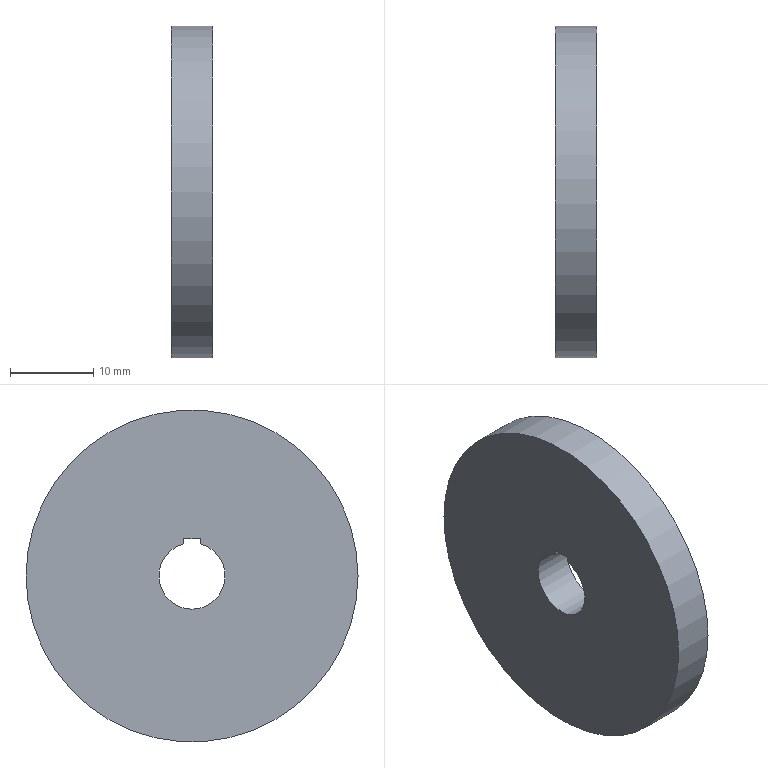Component | NX | SHE_JI-6 | 1 solid | 7 faces | box 5 x 40 x 40 mm | volume 6026 mm3 | plane 5 | cylinder 2 | commonest cylinder face diameters 40 x1 8 x1
STEP:
#1=CARTESIAN_POINT('',(0.,0.,0.));
#2=DIRECTION('',(0.,0.,1.));
#3=DIRECTION('',(1.,0.,0.));
#4=AXIS2_PLACEMENT_3D('',#1,#2,#3);
#5=CARTESIAN_POINT('',(-21.06,-1.,40.5));
#6=VERTEX_POINT('',#5);
#7=CARTESIAN_POINT('',(-21.06,-1.,39.873));
#8=VERTEX_POINT('',#7);
#9=CARTESIAN_POINT('',(-21.06,-1.,36.));
#10=DIRECTION('',(0.,-0.,-1.));
#11=VECTOR('',#10,1.);
#12=LINE('',#9,#11);
#13=CARTESIAN_POINT('',(-21.06,-0.,36.));
#14=DIRECTION('',(1.,0.,0.));
#15=DIRECTION('',(0.,1.,0.));
#16=AXIS2_PLACEMENT_3D('',#13,#14,#15);
#17=PLANE('',#16);
#18=CARTESIAN_POINT('',(-1.,0.));
#19=DIRECTION('',(-0.,-1.));
#20=VECTOR('',#19,1.);
#21=LINE('',#18,#20);
#22=(GEOMETRIC_REPRESENTATION_CONTEXT(2)PARAMETRIC_REPRESENTATION_CONTEXT()REPRESENTATION_CONTEXT('',''));
#23=DEFINITIONAL_REPRESENTATION('',(#21),#22);
#24=PCURVE('',#17,#23);
#25=CARTESIAN_POINT('',(-31.06,-1.,40.5));
#26=DIRECTION('',(0.,-1.,0.));
#27=DIRECTION('',(0.,-0.,-1.));
#28=AXIS2_PLACEMENT_3D('',#25,#26,#27);
#29=PLANE('',#28);
#30=CARTESIAN_POINT('',(4.5,10.));
#31=DIRECTION('',(1.,0.));
#32=VECTOR('',#31,1.);
#33=LINE('',#30,#32);
#34=(GEOMETRIC_REPRESENTATION_CONTEXT(2)PARAMETRIC_REPRESENTATION_CONTEXT()REPRESENTATION_CONTEXT('',''));
#35=DEFINITIONAL_REPRESENTATION('',(#33),#34);
#36=PCURVE('',#29,#35);
#37=SURFACE_CURVE('',#12,(#24,#36),.PCURVE_S1.);
#38=EDGE_CURVE('',#6,#8,#37,.T.);
#39=ORIENTED_EDGE('',*,*,#38,.F.);
#40=CARTESIAN_POINT('',(-21.06,1.,40.5));
#41=VERTEX_POINT('',#40);
#42=CARTESIAN_POINT('',(-21.06,-0.,40.5));
#43=DIRECTION('',(0.,-1.,-0.));
#44=VECTOR('',#43,1.);
#45=LINE('',#42,#44);
#46=CARTESIAN_POINT('',(-0.,4.5));
#47=DIRECTION('',(-1.,-0.));
#48=VECTOR('',#47,1.);
#49=LINE('',#46,#48);
#50=(GEOMETRIC_REPRESENTATION_CONTEXT(2)PARAMETRIC_REPRESENTATION_CONTEXT()REPRESENTATION_CONTEXT('',''));
#51=DEFINITIONAL_REPRESENTATION('',(#49),#50);
#52=PCURVE('',#17,#51);
#53=CARTESIAN_POINT('',(-31.06,1.,40.5));
#54=DIRECTION('',(0.,-0.,1.));
#55=DIRECTION('',(0.,-1.,-0.));
#56=AXIS2_PLACEMENT_3D('',#53,#54,#55);
#57=PLANE('',#56);
#58=CARTESIAN_POINT('',(1.,10.));
#59=DIRECTION('',(1.,0.));
#60=VECTOR('',#59,1.);
#61=LINE('',#58,#60);
#62=(GEOMETRIC_REPRESENTATION_CONTEXT(2)PARAMETRIC_REPRESENTATION_CONTEXT()REPRESENTATION_CONTEXT('',''));
#63=DEFINITIONAL_REPRESENTATION('',(#61),#62);
#64=PCURVE('',#57,#63);
#65=SURFACE_CURVE('',#45,(#52,#64),.PCURVE_S1.);
#66=EDGE_CURVE('',#41,#6,#65,.T.);
#67=ORIENTED_EDGE('',*,*,#66,.F.);
#68=CARTESIAN_POINT('',(-21.06,1.,39.873));
#69=VERTEX_POINT('',#68);
#70=CARTESIAN_POINT('',(-21.06,1.,36.));
#71=DIRECTION('',(0.,0.,1.));
#72=VECTOR('',#71,1.);
#73=LINE('',#70,#72);
#74=CARTESIAN_POINT('',(1.,0.));
#75=DIRECTION('',(0.,1.));
#76=VECTOR('',#75,1.);
#77=LINE('',#74,#76);
#78=(GEOMETRIC_REPRESENTATION_CONTEXT(2)PARAMETRIC_REPRESENTATION_CONTEXT()REPRESENTATION_CONTEXT('',''));
#79=DEFINITIONAL_REPRESENTATION('',(#77),#78);
#80=PCURVE('',#17,#79);
#81=CARTESIAN_POINT('',(-31.06,1.,36.7));
#82=DIRECTION('',(0.,1.,0.));
#83=DIRECTION('',(-1.,0.,0.));
#84=AXIS2_PLACEMENT_3D('',#81,#82,#83);
#85=PLANE('',#84);
#86=CARTESIAN_POINT('',(-10.,-0.7));
#87=DIRECTION('',(0.,1.));
#88=VECTOR('',#87,1.);
#89=LINE('',#86,#88);
#90=(GEOMETRIC_REPRESENTATION_CONTEXT(2)PARAMETRIC_REPRESENTATION_CONTEXT()REPRESENTATION_CONTEXT('',''));
#91=DEFINITIONAL_REPRESENTATION('',(#89),#90);
#92=PCURVE('',#85,#91);
#93=SURFACE_CURVE('',#73,(#80,#92),.PCURVE_S1.);
#94=EDGE_CURVE('',#69,#41,#93,.T.);
#95=ORIENTED_EDGE('',*,*,#94,.F.);
#96=CARTESIAN_POINT('',(-21.06,-0.,36.));
#97=DIRECTION('',(-1.,0.,0.));
#98=DIRECTION('',(0.,1.,-0.));
#99=AXIS2_PLACEMENT_3D('',#96,#97,#98);
#100=CIRCLE('',#99,4.);
#101=CARTESIAN_POINT('',(4.,-0.));
#102=CARTESIAN_POINT('',(4.,-6.928));
#103=CARTESIAN_POINT('',(-2.,-3.464));
#104=CARTESIAN_POINT('',(-8.,-0.));
#105=CARTESIAN_POINT('',(-2.,3.464));
#106=CARTESIAN_POINT('',(4.,6.928));
#107=CARTESIAN_POINT('',(4.,-0.));
#108=(BOUNDED_CURVE()B_SPLINE_CURVE(2,(#101,#102,#103,#104,#105,#106,#107),.UNSPECIFIED.,.T.,.F.)B_SPLINE_CURVE_WITH_KNOTS((1,2,2,2,2,1),(-2.094,0.,2.094,4.189,6.283,8.378),.UNSPECIFIED.)CURVE()GEOMETRIC_REPRESENTATION_ITEM()RATIONAL_B_SPLINE_CURVE((1.,0.5,1.,0.5,1.,0.5,1.))REPRESENTATION_ITEM(''));
#109=(GEOMETRIC_REPRESENTATION_CONTEXT(2)PARAMETRIC_REPRESENTATION_CONTEXT()REPRESENTATION_CONTEXT('',''));
#110=DEFINITIONAL_REPRESENTATION('',(#108),#109);
#111=PCURVE('',#17,#110);
#112=CARTESIAN_POINT('',(-21.06,-0.,36.));
#113=DIRECTION('',(-1.,0.,0.));
#114=DIRECTION('',(0.,1.,-0.));
#115=AXIS2_PLACEMENT_3D('',#112,#113,#114);
#116=CYLINDRICAL_SURFACE('',#115,4.);
#117=CARTESIAN_POINT('',(-6.283,0.));
#118=DIRECTION('',(1.,0.));
#119=VECTOR('',#118,1.);
#120=LINE('',#117,#119);
#121=(GEOMETRIC_REPRESENTATION_CONTEXT(2)PARAMETRIC_REPRESENTATION_CONTEXT()REPRESENTATION_CONTEXT('',''));
#122=DEFINITIONAL_REPRESENTATION('',(#120),#121);
#123=PCURVE('',#116,#122);
#124=SURFACE_CURVE('',#100,(#111,#123),.PCURVE_S1.);
#125=EDGE_CURVE('',#69,#8,#124,.T.);
#126=ORIENTED_EDGE('',*,*,#125,.T.);
#127=EDGE_LOOP('',(#39,#67,#95,#126));
#128=FACE_BOUND('',#127,.T.);
#129=CARTESIAN_POINT('',(-21.06,20.,36.));
#130=VERTEX_POINT('',#129);
#131=CARTESIAN_POINT('',(-21.06,-0.,36.));
#132=DIRECTION('',(-1.,0.,0.));
#133=DIRECTION('',(0.,1.,0.));
#134=AXIS2_PLACEMENT_3D('',#131,#132,#133);
#135=CIRCLE('',#134,20.);
#136=CARTESIAN_POINT('',(20.,0.));
#137=CARTESIAN_POINT('',(20.,-34.641));
#138=CARTESIAN_POINT('',(-10.,-17.321));
#139=CARTESIAN_POINT('',(-40.,-0.));
#140=CARTESIAN_POINT('',(-10.,17.321));
#141=CARTESIAN_POINT('',(20.,34.641));
#142=CARTESIAN_POINT('',(20.,0.));
#143=(BOUNDED_CURVE()B_SPLINE_CURVE(2,(#136,#137,#138,#139,#140,#141,#142),.UNSPECIFIED.,.T.,.F.)B_SPLINE_CURVE_WITH_KNOTS((1,2,2,2,2,1),(-2.094,0.,2.094,4.189,6.283,8.378),.UNSPECIFIED.)CURVE()GEOMETRIC_REPRESENTATION_ITEM()RATIONAL_B_SPLINE_CURVE((1.,0.5,1.,0.5,1.,0.5,1.))REPRESENTATION_ITEM(''));
#144=(GEOMETRIC_REPRESENTATION_CONTEXT(2)PARAMETRIC_REPRESENTATION_CONTEXT()REPRESENTATION_CONTEXT('',''));
#145=DEFINITIONAL_REPRESENTATION('',(#143),#144);
#146=PCURVE('',#17,#145);
#147=CARTESIAN_POINT('',(-26.06,-0.,36.));
#148=DIRECTION('',(1.,0.,0.));
#149=DIRECTION('',(0.,1.,0.));
#150=AXIS2_PLACEMENT_3D('',#147,#148,#149);
#151=CYLINDRICAL_SURFACE('',#150,20.);
#152=CARTESIAN_POINT('',(6.283,5.));
#153=DIRECTION('',(-1.,0.));
#154=VECTOR('',#153,1.);
#155=LINE('',#152,#154);
#156=(GEOMETRIC_REPRESENTATION_CONTEXT(2)PARAMETRIC_REPRESENTATION_CONTEXT()REPRESENTATION_CONTEXT('',''));
#157=DEFINITIONAL_REPRESENTATION('',(#155),#156);
#158=PCURVE('',#151,#157);
#159=SURFACE_CURVE('',#135,(#146,#158),.PCURVE_S1.);
#160=EDGE_CURVE('',#130,#130,#159,.T.);
#161=ORIENTED_EDGE('',*,*,#160,.F.);
#162=EDGE_LOOP('',(#161));
#163=FACE_BOUND('',#162,.T.);
#164=ADVANCED_FACE('',(#128,#163),#17,.T.);
#165=CARTESIAN_POINT('',(-26.06,-1.,39.873));
#166=VERTEX_POINT('',#165);
#167=CARTESIAN_POINT('',(-26.06,-1.,40.5));
#168=VERTEX_POINT('',#167);
#169=CARTESIAN_POINT('',(-26.06,-1.,36.));
#170=DIRECTION('',(0.,0.,1.));
#171=VECTOR('',#170,1.);
#172=LINE('',#169,#171);
#173=CARTESIAN_POINT('',(-26.06,-0.,36.));
#174=DIRECTION('',(-1.,0.,0.));
#175=DIRECTION('',(0.,-1.,0.));
#176=AXIS2_PLACEMENT_3D('',#173,#174,#175);
#177=PLANE('',#176);
#178=CARTESIAN_POINT('',(1.,0.));
#179=DIRECTION('',(-0.,1.));
#180=VECTOR('',#179,1.);
#181=LINE('',#178,#180);
#182=(GEOMETRIC_REPRESENTATION_CONTEXT(2)PARAMETRIC_REPRESENTATION_CONTEXT()REPRESENTATION_CONTEXT('',''));
#183=DEFINITIONAL_REPRESENTATION('',(#181),#182);
#184=PCURVE('',#177,#183);
#185=CARTESIAN_POINT('',(4.5,5.));
#186=DIRECTION('',(-1.,0.));
#187=VECTOR('',#186,1.);
#188=LINE('',#185,#187);
#189=(GEOMETRIC_REPRESENTATION_CONTEXT(2)PARAMETRIC_REPRESENTATION_CONTEXT()REPRESENTATION_CONTEXT('',''));
#190=DEFINITIONAL_REPRESENTATION('',(#188),#189);
#191=PCURVE('',#29,#190);
#192=SURFACE_CURVE('',#172,(#184,#191),.PCURVE_S1.);
#193=EDGE_CURVE('',#166,#168,#192,.T.);
#194=ORIENTED_EDGE('',*,*,#193,.F.);
#195=CARTESIAN_POINT('',(-26.06,1.,39.873));
#196=VERTEX_POINT('',#195);
#197=CARTESIAN_POINT('',(-26.06,0.,36.));
#198=DIRECTION('',(-1.,0.,0.));
#199=DIRECTION('',(0.,-1.,0.));
#200=AXIS2_PLACEMENT_3D('',#197,#198,#199);
#201=CIRCLE('',#200,4.);
#202=CARTESIAN_POINT('',(-0.,0.));
#203=DIRECTION('',(1.,0.));
#204=AXIS2_PLACEMENT_2D('',#202,#203);
#205=CIRCLE('',#204,4.);
#206=(GEOMETRIC_REPRESENTATION_CONTEXT(2)PARAMETRIC_REPRESENTATION_CONTEXT()REPRESENTATION_CONTEXT('',''));
#207=DEFINITIONAL_REPRESENTATION('',(#205),#206);
#208=PCURVE('',#177,#207);
#209=CARTESIAN_POINT('',(-3.142,5.));
#210=DIRECTION('',(1.,0.));
#211=VECTOR('',#210,1.);
#212=LINE('',#209,#211);
#213=(GEOMETRIC_REPRESENTATION_CONTEXT(2)PARAMETRIC_REPRESENTATION_CONTEXT()REPRESENTATION_CONTEXT('',''));
#214=DEFINITIONAL_REPRESENTATION('',(#212),#213);
#215=PCURVE('',#116,#214);
#216=SURFACE_CURVE('',#201,(#208,#215),.PCURVE_S1.);
#217=EDGE_CURVE('',#196,#166,#216,.T.);
#218=ORIENTED_EDGE('',*,*,#217,.F.);
#219=CARTESIAN_POINT('',(-26.06,1.,40.5));
#220=VERTEX_POINT('',#219);
#221=CARTESIAN_POINT('',(-26.06,1.,36.));
#222=DIRECTION('',(0.,0.,-1.));
#223=VECTOR('',#222,1.);
#224=LINE('',#221,#223);
#225=CARTESIAN_POINT('',(-1.,0.));
#226=DIRECTION('',(0.,-1.));
#227=VECTOR('',#226,1.);
#228=LINE('',#225,#227);
#229=(GEOMETRIC_REPRESENTATION_CONTEXT(2)PARAMETRIC_REPRESENTATION_CONTEXT()REPRESENTATION_CONTEXT('',''));
#230=DEFINITIONAL_REPRESENTATION('',(#228),#229);
#231=PCURVE('',#177,#230);
#232=CARTESIAN_POINT('',(-5.,-0.7));
#233=DIRECTION('',(0.,-1.));
#234=VECTOR('',#233,1.);
#235=LINE('',#232,#234);
#236=(GEOMETRIC_REPRESENTATION_CONTEXT(2)PARAMETRIC_REPRESENTATION_CONTEXT()REPRESENTATION_CONTEXT('',''));
#237=DEFINITIONAL_REPRESENTATION('',(#235),#236);
#238=PCURVE('',#85,#237);
#239=SURFACE_CURVE('',#224,(#231,#238),.PCURVE_S1.);
#240=EDGE_CURVE('',#220,#196,#239,.T.);
#241=ORIENTED_EDGE('',*,*,#240,.F.);
#242=CARTESIAN_POINT('',(-26.06,-0.,40.5));
#243=DIRECTION('',(0.,1.,0.));
#244=VECTOR('',#243,1.);
#245=LINE('',#242,#244);
#246=CARTESIAN_POINT('',(0.,4.5));
#247=DIRECTION('',(-1.,0.));
#248=VECTOR('',#247,1.);
#249=LINE('',#246,#248);
#250=(GEOMETRIC_REPRESENTATION_CONTEXT(2)PARAMETRIC_REPRESENTATION_CONTEXT()REPRESENTATION_CONTEXT('',''));
#251=DEFINITIONAL_REPRESENTATION('',(#249),#250);
#252=PCURVE('',#177,#251);
#253=CARTESIAN_POINT('',(1.,5.));
#254=DIRECTION('',(-1.,0.));
#255=VECTOR('',#254,1.);
#256=LINE('',#253,#255);
#257=(GEOMETRIC_REPRESENTATION_CONTEXT(2)PARAMETRIC_REPRESENTATION_CONTEXT()REPRESENTATION_CONTEXT('',''));
#258=DEFINITIONAL_REPRESENTATION('',(#256),#257);
#259=PCURVE('',#57,#258);
#260=SURFACE_CURVE('',#245,(#252,#259),.PCURVE_S1.);
#261=EDGE_CURVE('',#168,#220,#260,.T.);
#262=ORIENTED_EDGE('',*,*,#261,.F.);
#263=EDGE_LOOP('',(#194,#218,#241,#262));
#264=FACE_BOUND('',#263,.T.);
#265=CARTESIAN_POINT('',(-26.06,20.,36.));
#266=VERTEX_POINT('',#265);
#267=CARTESIAN_POINT('',(-26.06,-0.,36.));
#268=DIRECTION('',(1.,0.,0.));
#269=DIRECTION('',(0.,1.,0.));
#270=AXIS2_PLACEMENT_3D('',#267,#268,#269);
#271=CIRCLE('',#270,20.);
#272=CARTESIAN_POINT('',(-20.,0.));
#273=CARTESIAN_POINT('',(-20.,34.641));
#274=CARTESIAN_POINT('',(10.,17.321));
#275=CARTESIAN_POINT('',(40.,0.));
#276=CARTESIAN_POINT('',(10.,-17.321));
#277=CARTESIAN_POINT('',(-20.,-34.641));
#278=CARTESIAN_POINT('',(-20.,0.));
#279=(BOUNDED_CURVE()B_SPLINE_CURVE(2,(#272,#273,#274,#275,#276,#277,#278),.UNSPECIFIED.,.T.,.F.)B_SPLINE_CURVE_WITH_KNOTS((1,2,2,2,2,1),(-2.094,0.,2.094,4.189,6.283,8.378),.UNSPECIFIED.)CURVE()GEOMETRIC_REPRESENTATION_ITEM()RATIONAL_B_SPLINE_CURVE((1.,0.5,1.,0.5,1.,0.5,1.))REPRESENTATION_ITEM(''));
#280=(GEOMETRIC_REPRESENTATION_CONTEXT(2)PARAMETRIC_REPRESENTATION_CONTEXT()REPRESENTATION_CONTEXT('',''));
#281=DEFINITIONAL_REPRESENTATION('',(#279),#280);
#282=PCURVE('',#177,#281);
#283=CARTESIAN_POINT('',(0.,0.));
#284=DIRECTION('',(1.,0.));
#285=VECTOR('',#284,1.);
#286=LINE('',#283,#285);
#287=(GEOMETRIC_REPRESENTATION_CONTEXT(2)PARAMETRIC_REPRESENTATION_CONTEXT()REPRESENTATION_CONTEXT('',''));
#288=DEFINITIONAL_REPRESENTATION('',(#286),#287);
#289=PCURVE('',#151,#288);
#290=SURFACE_CURVE('',#271,(#282,#289),.PCURVE_S1.);
#291=EDGE_CURVE('',#266,#266,#290,.T.);
#292=ORIENTED_EDGE('',*,*,#291,.F.);
#293=EDGE_LOOP('',(#292));
#294=FACE_BOUND('',#293,.T.);
#295=ADVANCED_FACE('',(#264,#294),#177,.T.);
#296=ORIENTED_EDGE('',*,*,#160,.T.);
#297=CARTESIAN_POINT('',(-26.06,20.,36.));
#298=CARTESIAN_POINT('',(-21.06,20.,36.));
#299=B_SPLINE_CURVE_WITH_KNOTS('',1,(#297,#298),.UNSPECIFIED.,.F.,.F.,(2,2),(0.,5.),.PIECEWISE_BEZIER_KNOTS.);
#300=CARTESIAN_POINT('',(0.,0.));
#301=DIRECTION('',(0.,1.));
#302=VECTOR('',#301,1.);
#303=LINE('',#300,#302);
#304=(GEOMETRIC_REPRESENTATION_CONTEXT(2)PARAMETRIC_REPRESENTATION_CONTEXT()REPRESENTATION_CONTEXT('',''));
#305=DEFINITIONAL_REPRESENTATION('',(#303),#304);
#306=PCURVE('',#151,#305);
#307=CARTESIAN_POINT('',(6.283,0.));
#308=DIRECTION('',(0.,1.));
#309=VECTOR('',#308,1.);
#310=LINE('',#307,#309);
#311=(GEOMETRIC_REPRESENTATION_CONTEXT(2)PARAMETRIC_REPRESENTATION_CONTEXT()REPRESENTATION_CONTEXT('',''));
#312=DEFINITIONAL_REPRESENTATION('',(#310),#311);
#313=PCURVE('',#151,#312);
#314=SEAM_CURVE('',#299,(#306,#313),.PCURVE_S1.);
#315=EDGE_CURVE('',#266,#130,#314,.T.);
#316=ORIENTED_EDGE('',*,*,#315,.F.);
#317=ORIENTED_EDGE('',*,*,#291,.T.);
#318=ORIENTED_EDGE('',*,*,#315,.T.);
#319=EDGE_LOOP('',(#296,#316,#317,#318));
#320=FACE_BOUND('',#319,.T.);
#321=ADVANCED_FACE('',(#320),#151,.T.);
#322=CARTESIAN_POINT('',(-21.06,1.,39.873));
#323=DIRECTION('',(-1.,0.,0.));
#324=VECTOR('',#323,1.);
#325=LINE('',#322,#324);
#326=CARTESIAN_POINT('',(-1.318,0.));
#327=DIRECTION('',(0.,1.));
#328=VECTOR('',#327,1.);
#329=LINE('',#326,#328);
#330=(GEOMETRIC_REPRESENTATION_CONTEXT(2)PARAMETRIC_REPRESENTATION_CONTEXT()REPRESENTATION_CONTEXT('',''));
#331=DEFINITIONAL_REPRESENTATION('',(#329),#330);
#332=PCURVE('',#116,#331);
#333=CARTESIAN_POINT('',(-10.,3.173));
#334=DIRECTION('',(1.,0.));
#335=VECTOR('',#334,1.);
#336=LINE('',#333,#335);
#337=(GEOMETRIC_REPRESENTATION_CONTEXT(2)PARAMETRIC_REPRESENTATION_CONTEXT()REPRESENTATION_CONTEXT('',''));
#338=DEFINITIONAL_REPRESENTATION('',(#336),#337);
#339=PCURVE('',#85,#338);
#340=SURFACE_CURVE('',#325,(#332,#339),.PCURVE_S1.);
#341=EDGE_CURVE('',#69,#196,#340,.T.);
#342=ORIENTED_EDGE('',*,*,#341,.F.);
#343=ORIENTED_EDGE('',*,*,#125,.T.);
#344=CARTESIAN_POINT('',(-21.06,-1.,39.873));
#345=DIRECTION('',(1.,-0.,-0.));
#346=VECTOR('',#345,1.);
#347=LINE('',#344,#346);
#348=CARTESIAN_POINT('',(4.46,0.));
#349=DIRECTION('',(0.,-1.));
#350=VECTOR('',#349,1.);
#351=LINE('',#348,#350);
#352=(GEOMETRIC_REPRESENTATION_CONTEXT(2)PARAMETRIC_REPRESENTATION_CONTEXT()REPRESENTATION_CONTEXT('',''));
#353=DEFINITIONAL_REPRESENTATION('',(#351),#352);
#354=PCURVE('',#116,#353);
#355=CARTESIAN_POINT('',(0.627,10.));
#356=DIRECTION('',(0.,1.));
#357=VECTOR('',#356,1.);
#358=LINE('',#355,#357);
#359=(GEOMETRIC_REPRESENTATION_CONTEXT(2)PARAMETRIC_REPRESENTATION_CONTEXT()REPRESENTATION_CONTEXT('',''));
#360=DEFINITIONAL_REPRESENTATION('',(#358),#359);
#361=PCURVE('',#29,#360);
#362=SURFACE_CURVE('',#347,(#354,#361),.PCURVE_S1.);
#363=EDGE_CURVE('',#166,#8,#362,.T.);
#364=ORIENTED_EDGE('',*,*,#363,.F.);
#365=ORIENTED_EDGE('',*,*,#217,.F.);
#366=EDGE_LOOP('',(#342,#343,#364,#365));
#367=FACE_BOUND('',#366,.F.);
#368=ADVANCED_FACE('',(#367),#116,.F.);
#369=ORIENTED_EDGE('',*,*,#38,.T.);
#370=ORIENTED_EDGE('',*,*,#363,.F.);
#371=ORIENTED_EDGE('',*,*,#193,.T.);
#372=CARTESIAN_POINT('',(-31.06,-1.,40.5));
#373=DIRECTION('',(-1.,0.,0.));
#374=VECTOR('',#373,1.);
#375=LINE('',#372,#374);
#376=CARTESIAN_POINT('',(0.,0.));
#377=DIRECTION('',(0.,-1.));
#378=VECTOR('',#377,1.);
#379=LINE('',#376,#378);
#380=(GEOMETRIC_REPRESENTATION_CONTEXT(2)PARAMETRIC_REPRESENTATION_CONTEXT()REPRESENTATION_CONTEXT('',''));
#381=DEFINITIONAL_REPRESENTATION('',(#379),#380);
#382=PCURVE('',#29,#381);
#383=CARTESIAN_POINT('',(2.,0.));
#384=DIRECTION('',(0.,-1.));
#385=VECTOR('',#384,1.);
#386=LINE('',#383,#385);
#387=(GEOMETRIC_REPRESENTATION_CONTEXT(2)PARAMETRIC_REPRESENTATION_CONTEXT()REPRESENTATION_CONTEXT('',''));
#388=DEFINITIONAL_REPRESENTATION('',(#386),#387);
#389=PCURVE('',#57,#388);
#390=SURFACE_CURVE('',#375,(#382,#389),.PCURVE_S1.);
#391=EDGE_CURVE('',#6,#168,#390,.T.);
#392=ORIENTED_EDGE('',*,*,#391,.F.);
#393=EDGE_LOOP('',(#369,#370,#371,#392));
#394=FACE_BOUND('',#393,.T.);
#395=ADVANCED_FACE('',(#394),#29,.F.);
#396=ORIENTED_EDGE('',*,*,#94,.T.);
#397=CARTESIAN_POINT('',(-31.06,1.,40.5));
#398=DIRECTION('',(-1.,0.,0.));
#399=VECTOR('',#398,1.);
#400=LINE('',#397,#399);
#401=CARTESIAN_POINT('',(0.,3.8));
#402=DIRECTION('',(1.,0.));
#403=VECTOR('',#402,1.);
#404=LINE('',#401,#403);
#405=(GEOMETRIC_REPRESENTATION_CONTEXT(2)PARAMETRIC_REPRESENTATION_CONTEXT()REPRESENTATION_CONTEXT('',''));
#406=DEFINITIONAL_REPRESENTATION('',(#404),#405);
#407=PCURVE('',#85,#406);
#408=CARTESIAN_POINT('',(0.,0.));
#409=DIRECTION('',(0.,-1.));
#410=VECTOR('',#409,1.);
#411=LINE('',#408,#410);
#412=(GEOMETRIC_REPRESENTATION_CONTEXT(2)PARAMETRIC_REPRESENTATION_CONTEXT()REPRESENTATION_CONTEXT('',''));
#413=DEFINITIONAL_REPRESENTATION('',(#411),#412);
#414=PCURVE('',#57,#413);
#415=SURFACE_CURVE('',#400,(#407,#414),.PCURVE_S1.);
#416=EDGE_CURVE('',#41,#220,#415,.T.);
#417=ORIENTED_EDGE('',*,*,#416,.T.);
#418=ORIENTED_EDGE('',*,*,#240,.T.);
#419=ORIENTED_EDGE('',*,*,#341,.F.);
#420=EDGE_LOOP('',(#396,#417,#418,#419));
#421=FACE_BOUND('',#420,.T.);
#422=ADVANCED_FACE('',(#421),#85,.F.);
#423=ORIENTED_EDGE('',*,*,#66,.T.);
#424=ORIENTED_EDGE('',*,*,#391,.T.);
#425=ORIENTED_EDGE('',*,*,#261,.T.);
#426=ORIENTED_EDGE('',*,*,#416,.F.);
#427=EDGE_LOOP('',(#423,#424,#425,#426));
#428=FACE_BOUND('',#427,.T.);
#429=ADVANCED_FACE('',(#428),#57,.F.);
#430=CLOSED_SHELL('',(#164,#295,#321,#368,#395,#422,#429));
#431=MANIFOLD_SOLID_BREP('',#430);
#432=(LENGTH_UNIT()NAMED_UNIT(*)SI_UNIT(.MILLI.,.METRE.));
#433=UNCERTAINTY_MEASURE_WITH_UNIT(LENGTH_MEASURE(0.000002),#432,'','');
#434=(NAMED_UNIT(*)PLANE_ANGLE_UNIT()SI_UNIT($,.RADIAN.));
#435=(NAMED_UNIT(*)SI_UNIT($,.STERADIAN.)SOLID_ANGLE_UNIT());
#436=(GEOMETRIC_REPRESENTATION_CONTEXT(3)GLOBAL_UNCERTAINTY_ASSIGNED_CONTEXT((#433))GLOBAL_UNIT_ASSIGNED_CONTEXT((#432,#434,#435))REPRESENTATION_CONTEXT('',''));
#437=ADVANCED_BREP_SHAPE_REPRESENTATION('',(#4,#431),#436);